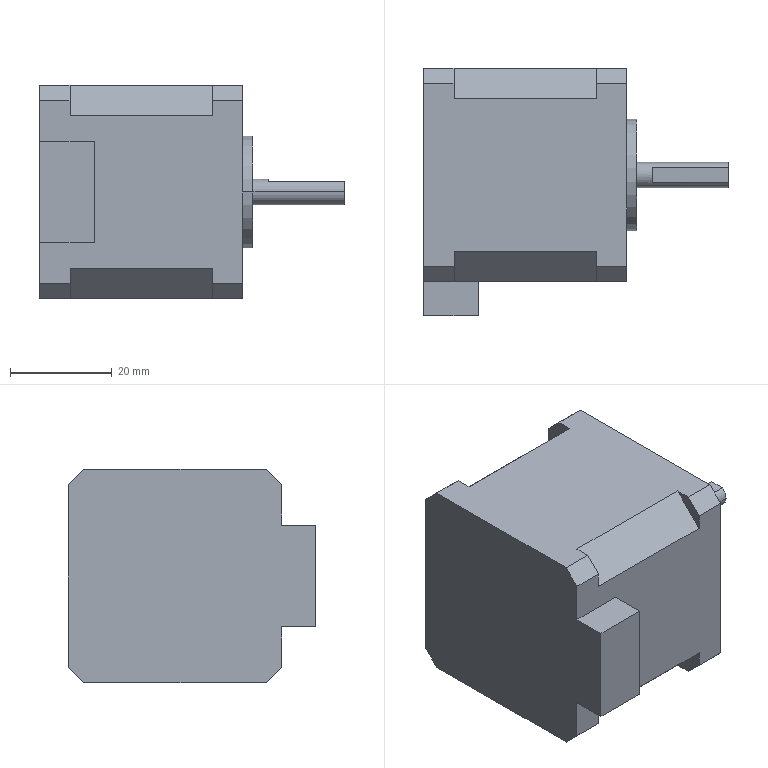Component | SolidWorks | Handball42-40Stepping-1 | 1 solid | 54 faces | box 60 x 48.7 x 42 mm | volume 70721 mm3 | plane 34 | cylinder 12 | cone 8 | commonest cylinder face diameters 2.5 x8 5 x2 22 x2
build123d program:
from build123d import *

# Parameters (mm, degrees)
SKETCH1_W             = 42
SKETCH1_H             = 42
BOSS_EXTRUDE1_DEPTH   = 40
M3_TAPPED_HOLE1_D     = 2.5
M3_TAPPED_HOLE1_DEPTH = 7.5
M3_TAPPED_HOLE1_TIP   = 0.7511
SKETCH9_W             = 6.7
SKETCH9_H             = 20
BOSS_EXTRUDE2_DEPTH   = 10.8
CUT_EXTRUDE1_DEPTH    = 28
CHAMFER1_SIZE         = 3
SKETCH11_R            = 11
BOSS_EXTRUDE3_DEPTH   = 2
SKETCH12_R            = 2.5
BOSS_EXTRUDE4_DEPTH   = 18
CUT_EXTRUDE2_START    = -15
CUT_EXTRUDE2_DEPTH    = 15


with BuildPart() as part:
    # Sketch1 → Boss-Extrude1 (new body)
    with BuildSketch(Plane.XY):
        Rectangle(SKETCH1_W, SKETCH1_H)
    extrude(amount=BOSS_EXTRUDE1_DEPTH)

    # M3 Tapped Hole1
    with Locations(Plane(origin=(0, 0, 0), x_dir=(-1, 0, 0), z_dir=(0, 0, -1))):
        with Locations((15.5, 15.5), (-15.5, 15.5), (-15.5, -15.5), (15.5, -15.5)):
            Hole(M3_TAPPED_HOLE1_D / 2, depth=M3_TAPPED_HOLE1_DEPTH)
            with Locations((0, 0, -(M3_TAPPED_HOLE1_DEPTH + M3_TAPPED_HOLE1_TIP / 2))):  # 118° drill point
                Cone(0, M3_TAPPED_HOLE1_D / 2, M3_TAPPED_HOLE1_TIP, mode=Mode.SUBTRACT)

    # Sketch9 → Boss-Extrude2 (add)
    with BuildSketch(Plane.XY.offset(40)):
        with Locations((-24.35, 0)):
            Rectangle(SKETCH9_W, SKETCH9_H)
    extrude(amount=-BOSS_EXTRUDE2_DEPTH)

    # Sketch10 → Cut-Extrude1 (cut)
    with BuildSketch(Plane(origin=(0, 0, 6), x_dir=(-1, 0, 0), z_dir=(0, 0, -1))):
        Polygon((21, -21), (15, -21), (21, -15), align=None)
        Polygon((-15, -21), (-21, -15), (-21, -21), align=None)
        Polygon((-21, 15), (-15, 21), (-21, 21), align=None)
        Polygon((15, 21), (21, 15), (21, 21), align=None)
    extrude(amount=-CUT_EXTRUDE1_DEPTH, mode=Mode.SUBTRACT)

    # Chamfer1
    chamfer1_edges = [part.edges().sort_by_distance(p)[0] for p in [
        (-21, 21, 37),
        (-21, -21, 37),
        (21, -21, 37),
        (21, 21, 37),
        (21, 21, 3),
        (21, -21, 3),
        (-21, -21, 3),
        (-21, 21, 3),
    ]]
    chamfer(chamfer1_edges, length=CHAMFER1_SIZE)

    # Sketch11 → Boss-Extrude3 (add)
    with BuildSketch(Plane(origin=(0, 0, 0), x_dir=(-1, 0, 0), z_dir=(0, 0, -1))):
        with Locations(Location((0, 0, 0), (0, 0, 180))):
            Circle(SKETCH11_R)
    extrude(amount=BOSS_EXTRUDE3_DEPTH)

    # Sketch12 → Boss-Extrude4 (add)
    with BuildSketch(Plane(origin=(0, 0, -2), x_dir=(-1, 0, 0), z_dir=(0, 0, -1))):
        Circle(SKETCH12_R)
    extrude(amount=BOSS_EXTRUDE4_DEPTH)

    # Sketch13 → Cut-Extrude2 (cut)
    with BuildSketch(Plane(origin=(0, 0, -20), x_dir=(-1, 0, 0), z_dir=(0, 0, -1)).offset(CUT_EXTRUDE2_START)):
        with BuildLine():
            Line((1.5, -2), (-1.5, -2))
            ThreePointArc((-1.5, -2), (0, -2.5), (1.5, -2))
        make_face()
    extrude(amount=CUT_EXTRUDE2_DEPTH, mode=Mode.SUBTRACT)


solid = part.part

# Placed as in the assembly
solid = solid.moved(Location((-29.695, -5.355, -97.449), (-90, -90, 0)))